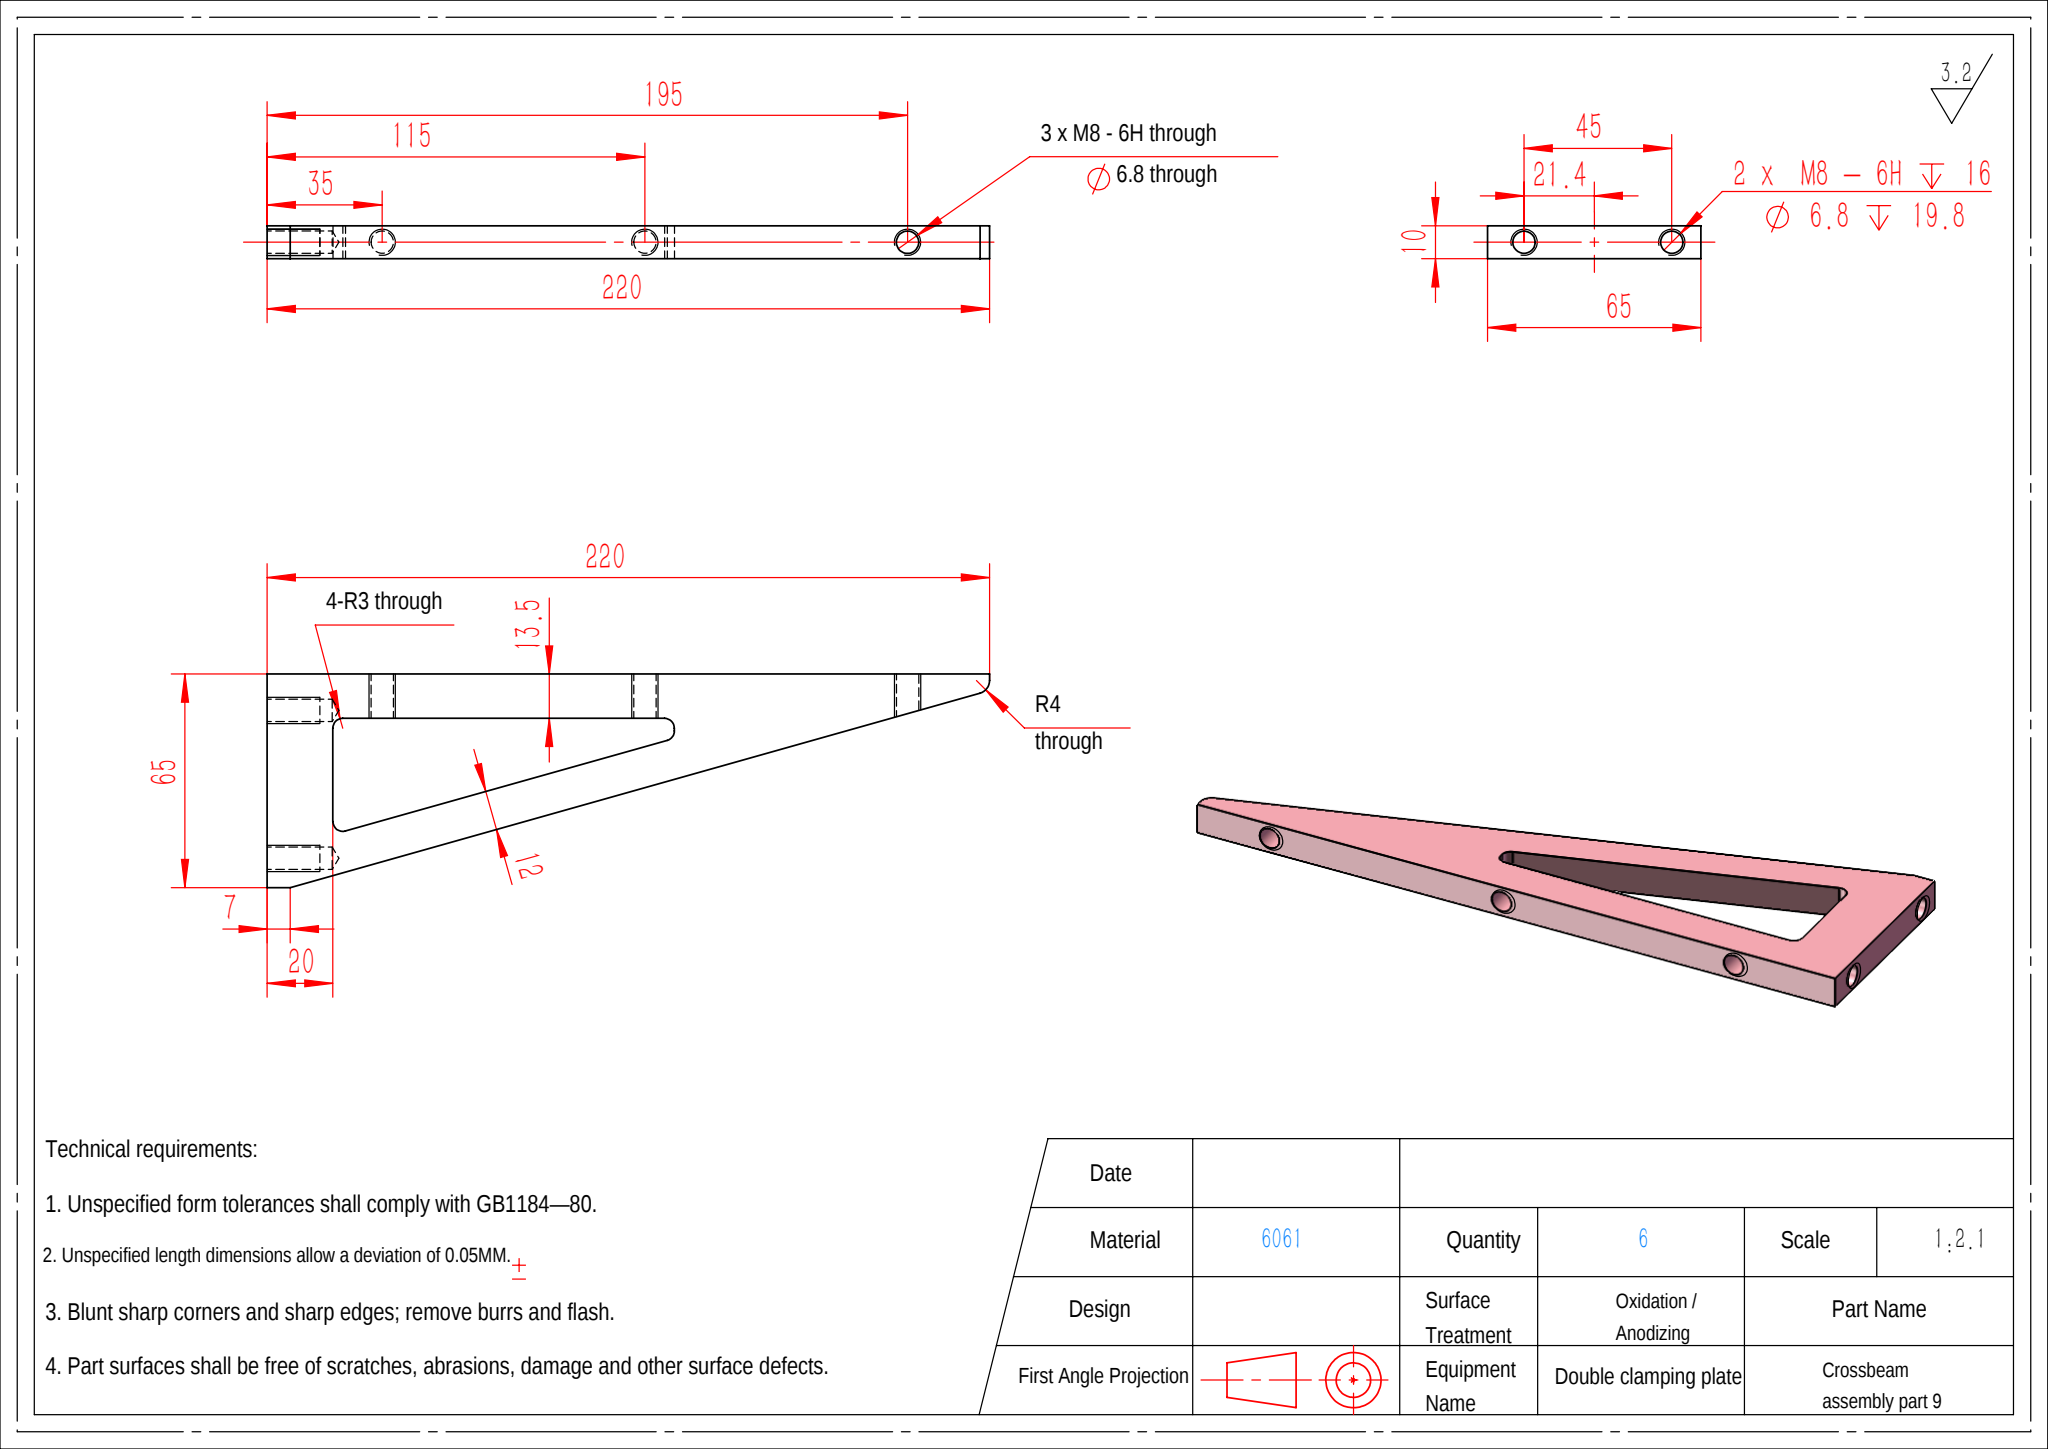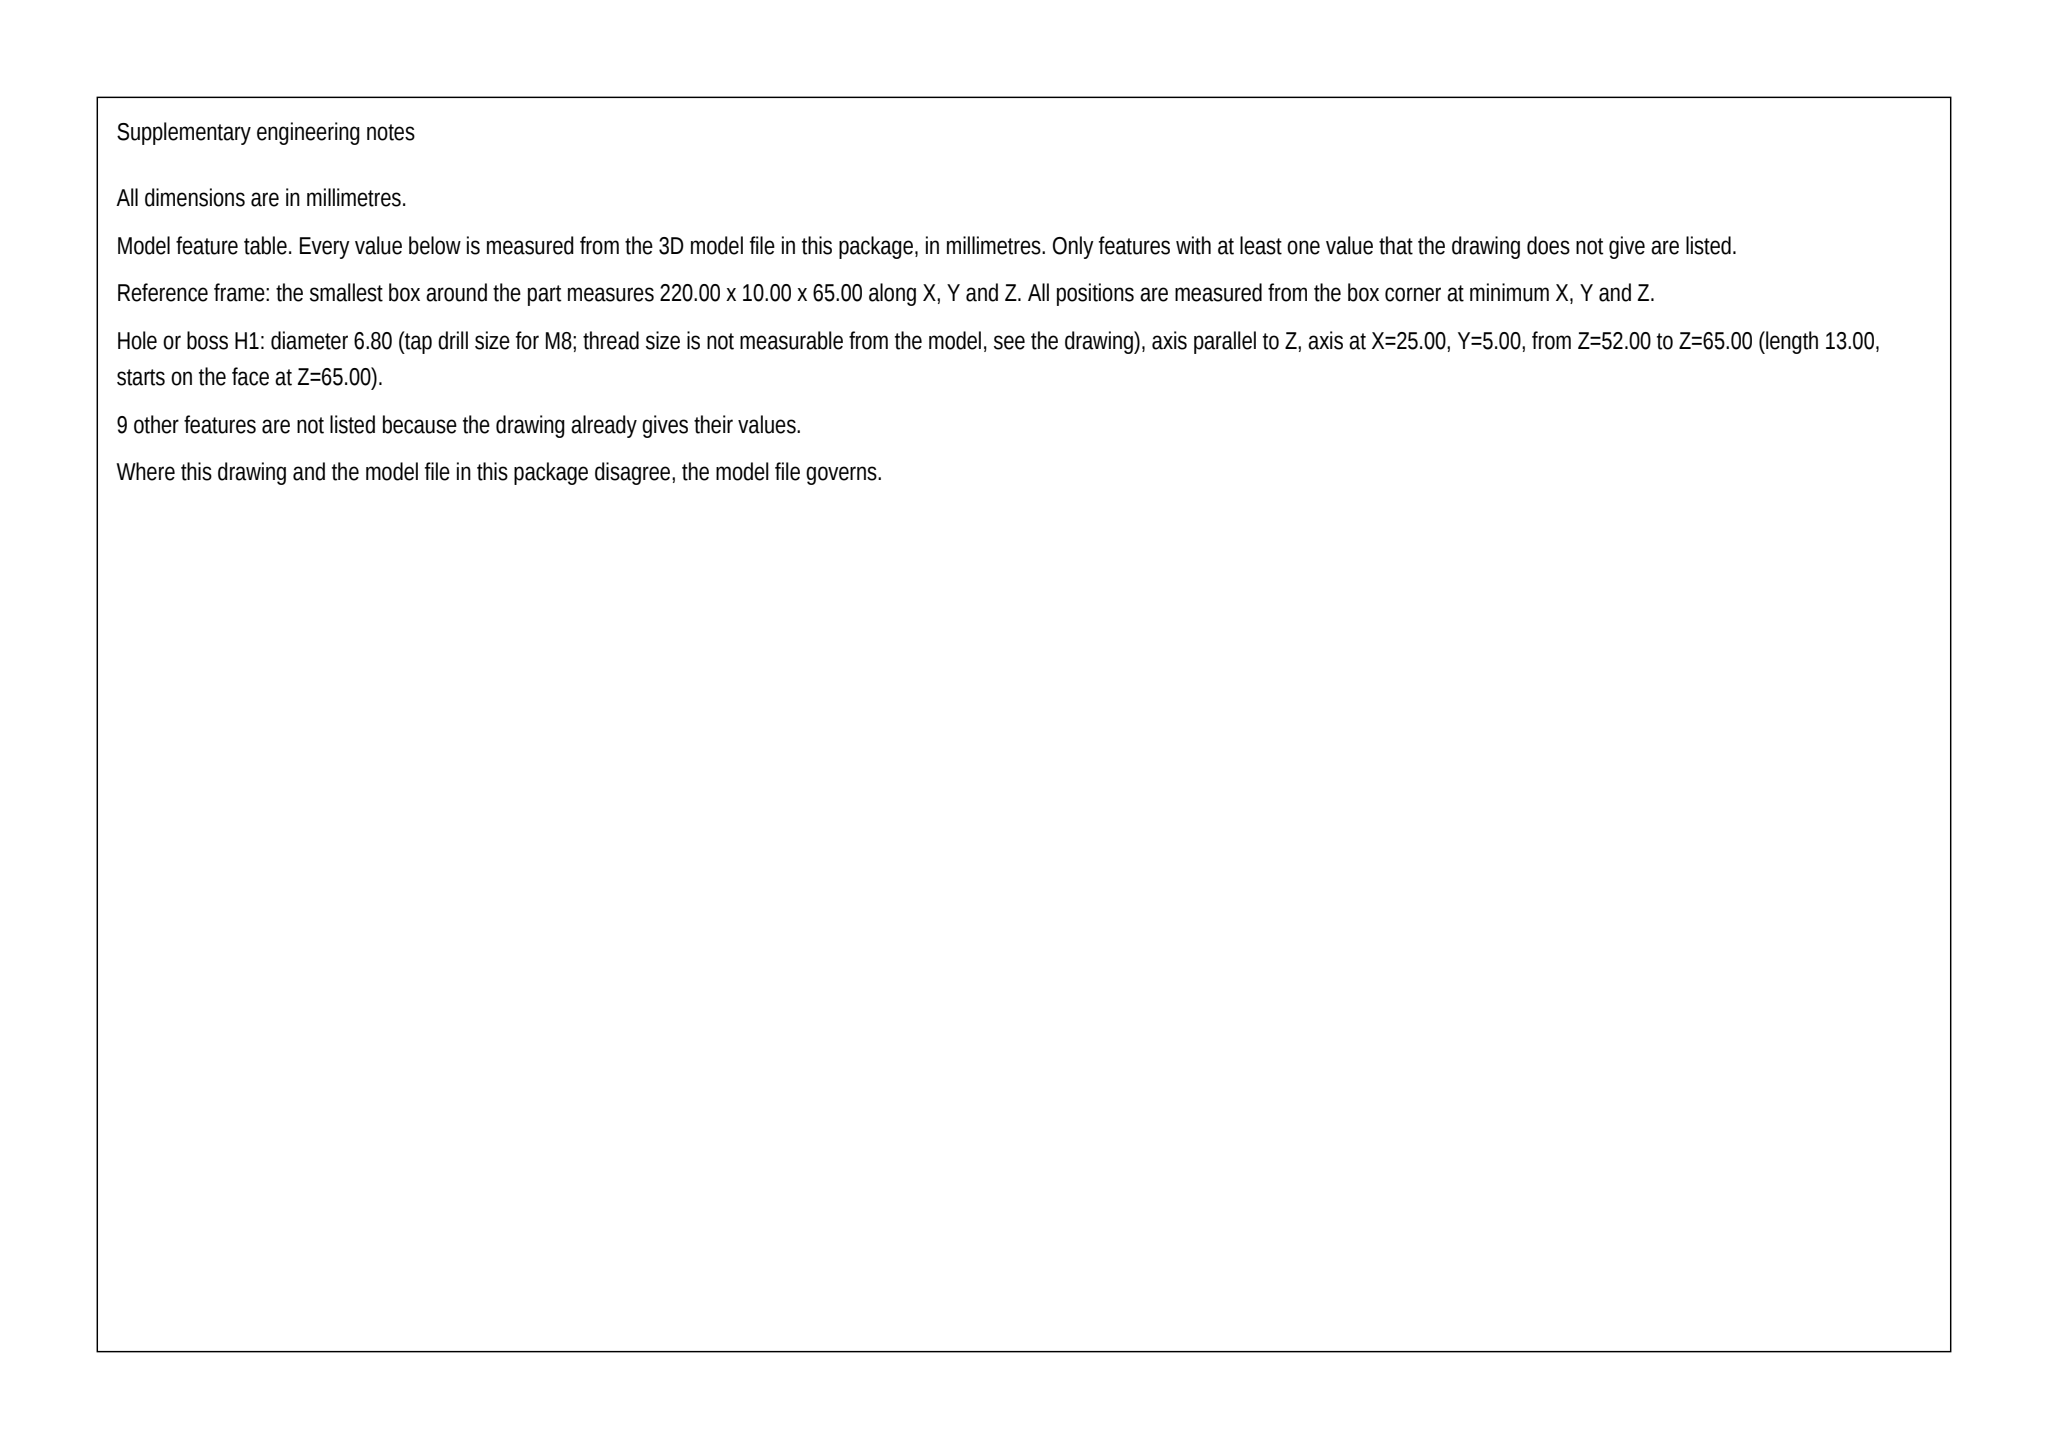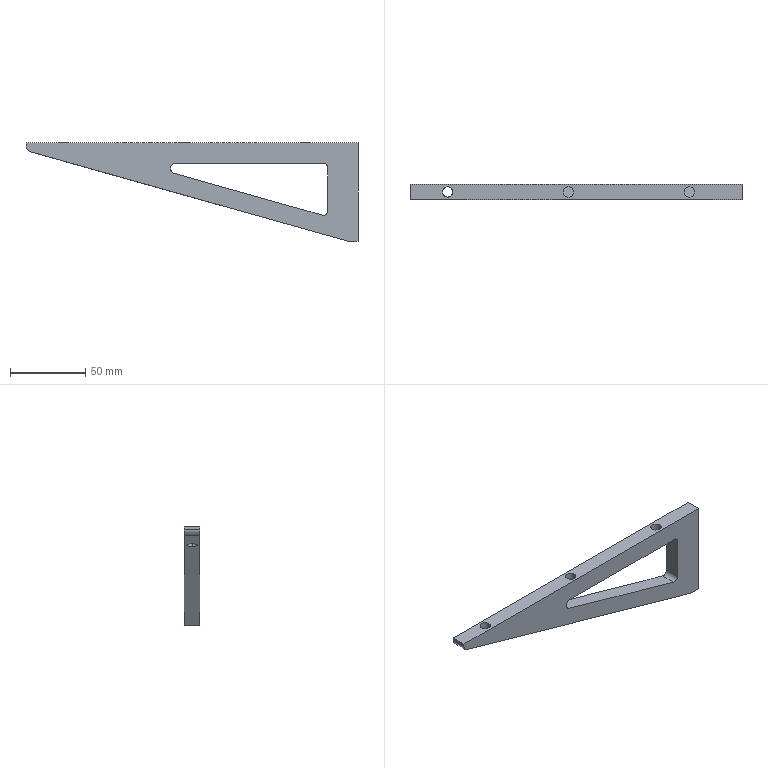Part | SolidWorks | mm | material 6061 | 1 solid | 30 faces | box 220 x 10 x 65 mm | volume 54713 mm3 | cylinder 15 | plane 11 | cone 4 | commonest cylinder face diameters 6.8 x10 6 x4 8 x1
build123d program:
from build123d import *

# Parameters (mm, degrees)
BOSS_EXTRUDE1_DEPTH   = 10
CUT_EXTRUDE1_DEPTH    = 230.619
M8_TAPPED_HOLE2_D     = 6.8
M8_TAPPED_HOLE2_DEPTH = 13.5
M8_TAPPED_HOLE1_D     = 6.8
M8_TAPPED_HOLE1_DEPTH = 19.75
M8_TAPPED_HOLE1_TIP   = 2.043
FILLET1_R             = 3
FILLET2_R             = 4
LPATTERN1_COUNT       = 3
LPATTERN1_PITCH       = 80


with BuildPart() as part:
    # Sketch1 → Boss-Extrude1 (new body)
    with BuildSketch(Plane.XZ):
        Polygon((0, 0), (0, -5), (213, -65), (220, -65), (220, 0), align=None)
    extrude(amount=-BOSS_EXTRUDE1_DEPTH)

    # Sketch2 → Cut-Extrude1 (cut, through all)
    with BuildSketch(Plane(origin=(0, 10, 0), x_dir=(-1, 0, 0), z_dir=(0, 1, 0))):
        with BuildLine():
            Line((-96, -19.575), (-96, -13.5))
            Line((-96, -13.5), (-197, -13.5))
            ThreePointArc((-197, -13.5), (-199.121, -14.379), (-200, -16.5))
            Line((-200, -16.5), (-200, -44.909))
            ThreePointArc((-200, -44.909), (-198.811, -47.301), (-196.187, -47.797))
            Line((-196.187, -47.797), (-96, -19.575))
        make_face()
    extrude(amount=-CUT_EXTRUDE1_DEPTH, mode=Mode.SUBTRACT)

    # M8 Tapped Hole2
    with Locations(Plane.XY):
        with Locations((185, 5)):
            m8_tapped_hole2 = Hole(M8_TAPPED_HOLE2_D / 2, depth=M8_TAPPED_HOLE2_DEPTH)

    # M8 Tapped Hole1
    with Locations(Plane(origin=(220, 0, 0), x_dir=(0, 0, -1), z_dir=(1, 0, 0))):
        with Locations((11.1, 5), (56.1, 5)):
            Hole(M8_TAPPED_HOLE1_D / 2, depth=M8_TAPPED_HOLE1_DEPTH)
            with Locations((0, 0, -(M8_TAPPED_HOLE1_DEPTH + M8_TAPPED_HOLE1_TIP / 2))):  # 118° drill point
                Cone(0, M8_TAPPED_HOLE1_D / 2, M8_TAPPED_HOLE1_TIP, mode=Mode.SUBTRACT)

    # Fillet1
    fillet1_edges = [part.edges().sort_by_distance(p)[0] for p in [
        (96, 5, -19.575),
        (96, 5, -13.5),
    ]]
    fillet(fillet1_edges, radius=FILLET1_R)

    # Fillet2
    fillet2_edges = [part.edges().sort_by_distance(p)[0] for p in [
        (0, 5, -5),
    ]]
    fillet(fillet2_edges, radius=FILLET2_R)

    # LPattern1: M8 Tapped Hole2 ×3
    with Locations(*[(-i * LPATTERN1_PITCH, 0, 0) for i in range(1, LPATTERN1_COUNT)]):
        add(m8_tapped_hole2, mode=Mode.SUBTRACT)


solid = part.part